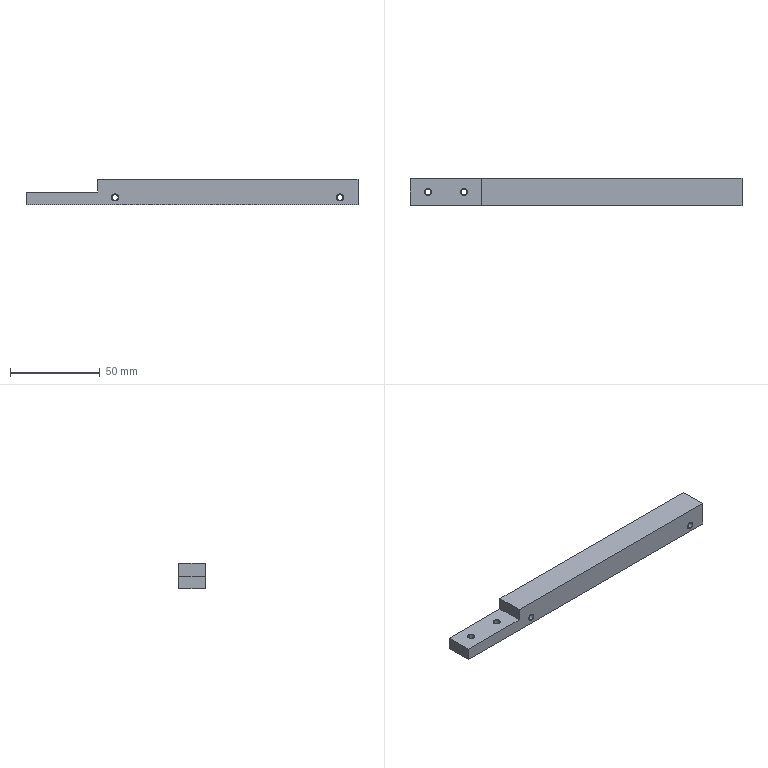CAM job | Mastercam | mm | 11 operations | part box 184.5 x 15 x 14
1. Facing | 24 - 50 平铣刀
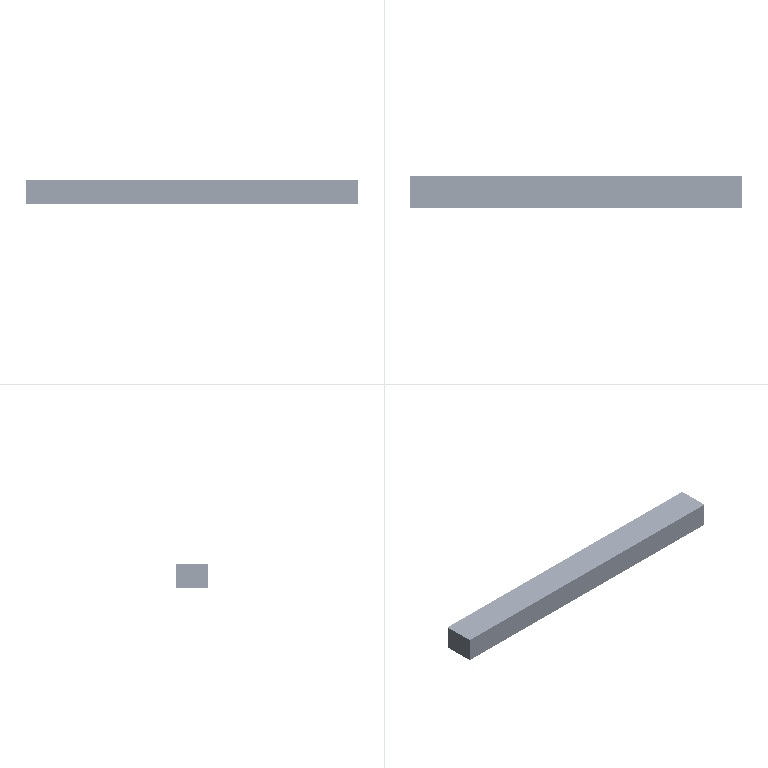2. Contour (Ramp) | 10 - 10 平铣刀
3. Contour (2D) | 8 - 8 平铣刀
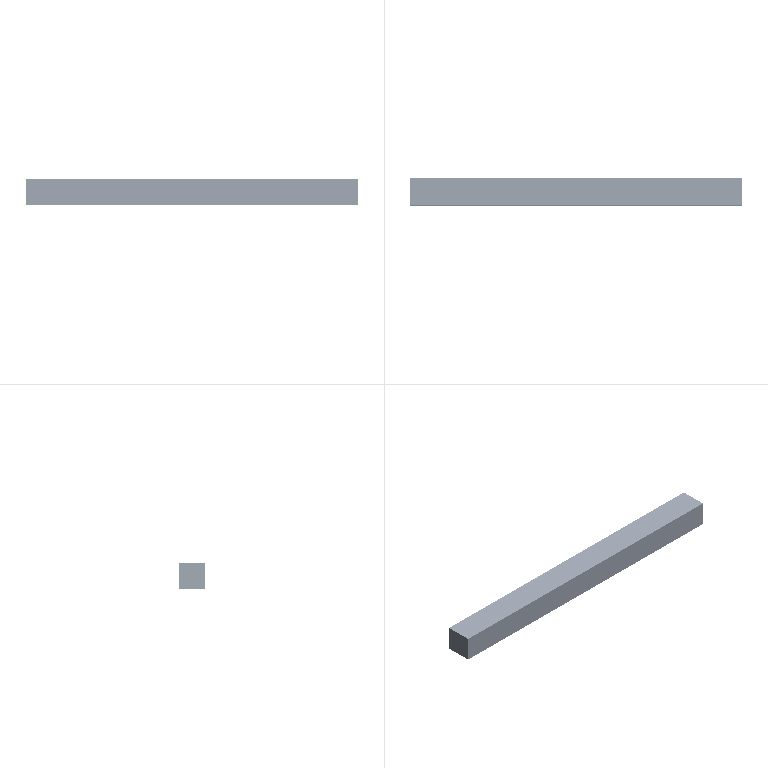4. Contour (2D chamfer) | 7 - 6 倒角刀
5. Facing | 24 - 50 平铣刀
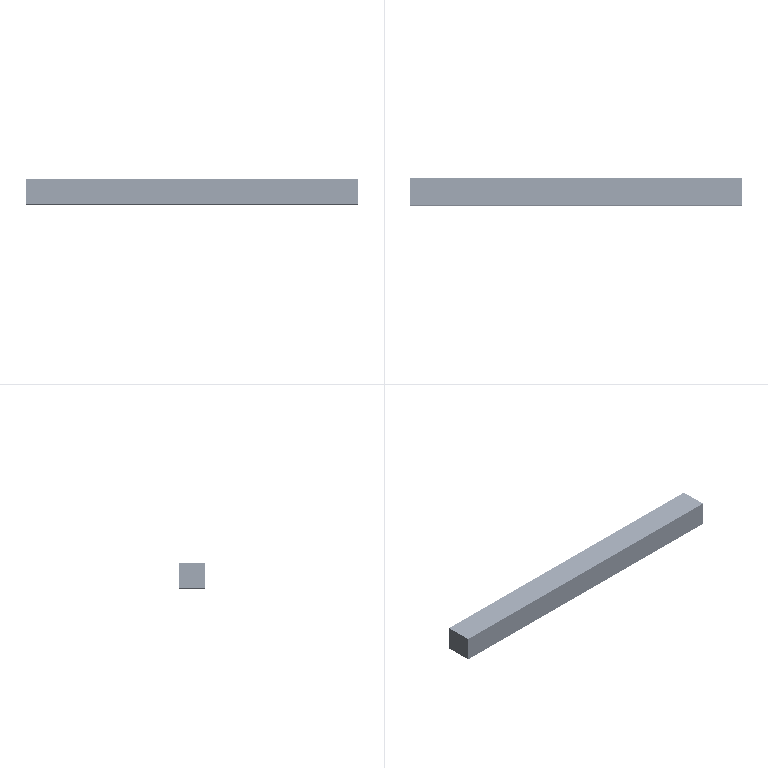6. Contour (Ramp) | 10 - 10 平铣刀
7. Contour (2D) | 10 - 10 平铣刀
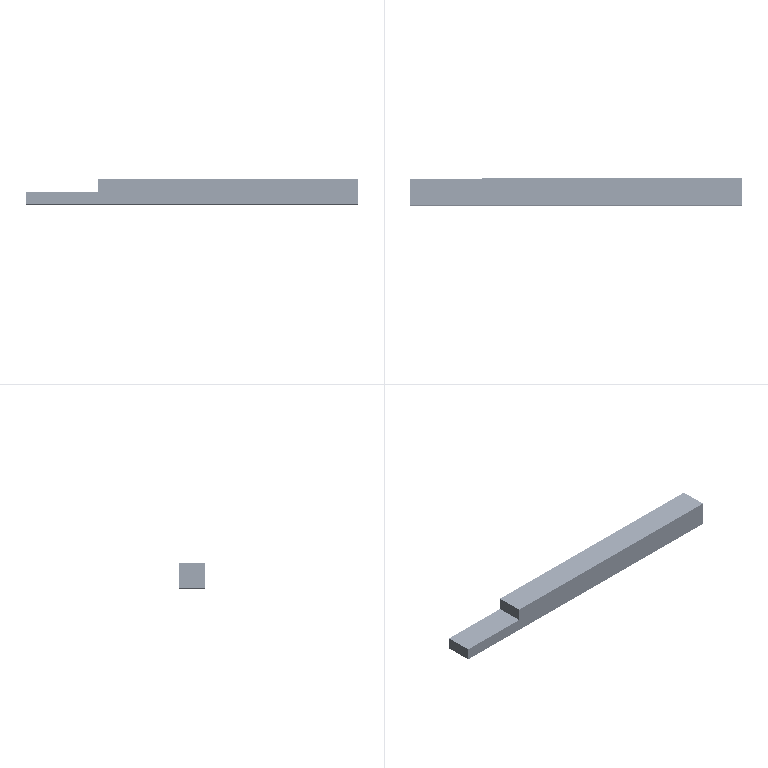8. Drill/Counterbore | 7 - 6 倒角刀
9. Contour (2D chamfer) | 7 - 6 倒角刀
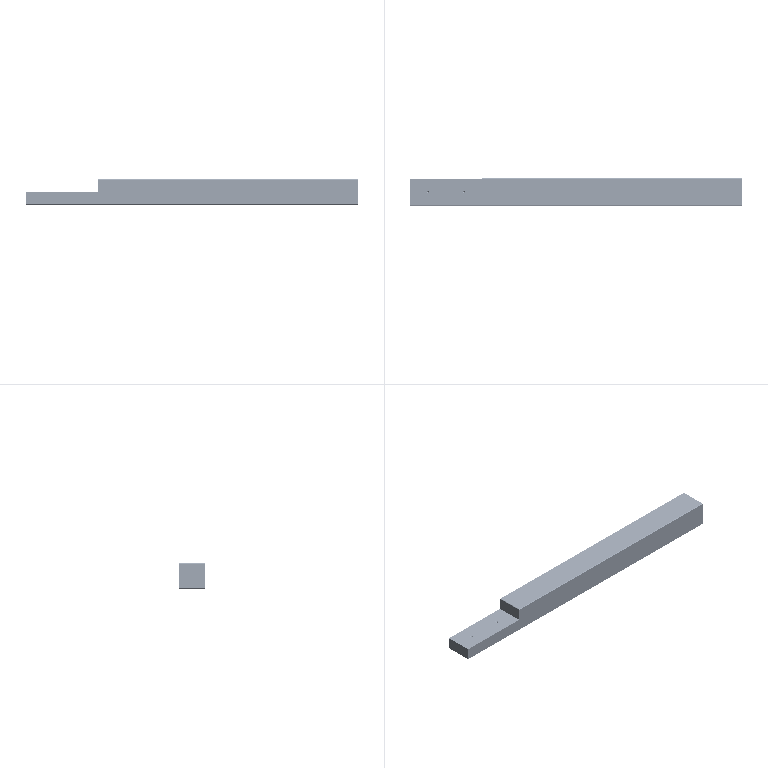10. Contour (2D chamfer) | 7 - 6 倒角刀
11. Drill/Counterbore | 7 - 6 倒角刀